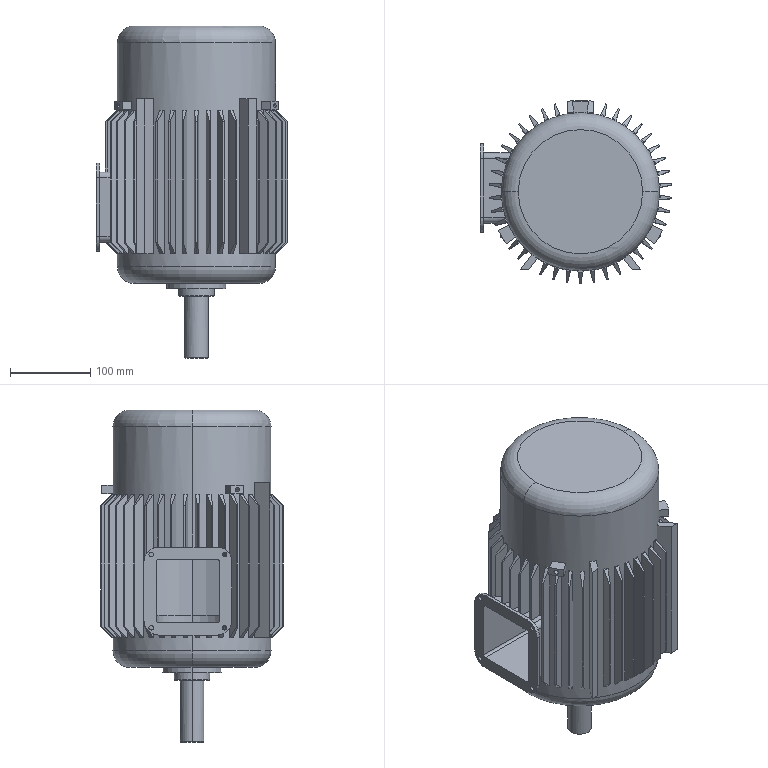Component | SolidWorks | Three-PhaseAsynchronousMotor-1_Motor-1 | 1 solid | 399 faces | volume 7077486 mm3 | plane 213 | cylinder 92 | cone 90 | torus 4 | commonest cylinder face diameters 227.5 x43 5.6 x12 5.775 x6 14 x4 36.4 x4 225.4 x3 196.7 x2 73.5 x2